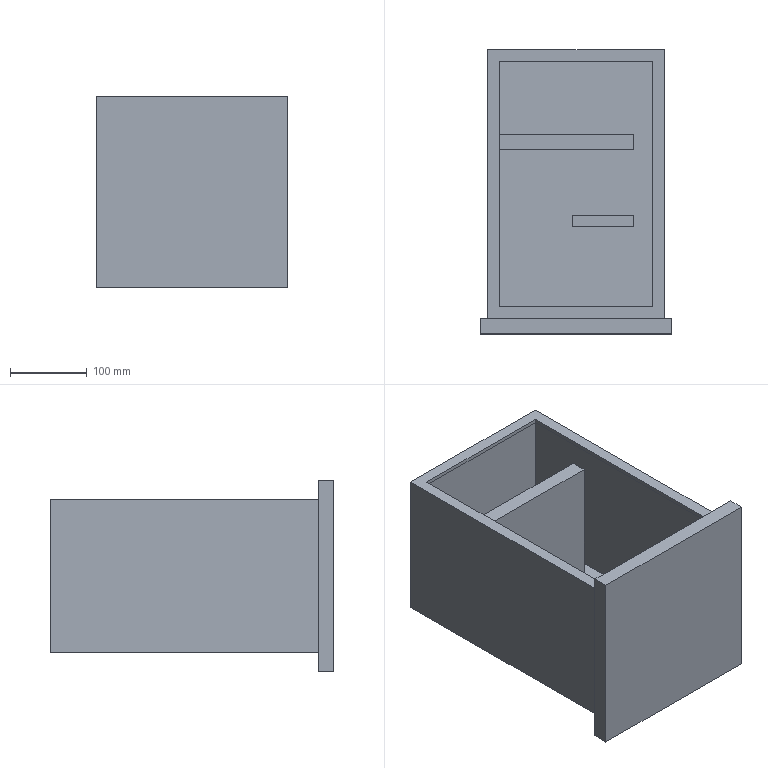Component | SolidWorks | ElectricalCabinet-2 | 1 solid | 30 faces | box 250 x 370 x 250 mm | volume 4917500 mm3 | plane 30
build123d program:
from build123d import *

# Parameters (mm, degrees)
SKETCH1_W           = 350
SKETCH1_H           = 200
BOSS_EXTRUDE1_DEPTH = 230
SHELL1_T            = -10
SKETCH2_W           = 350
SKETCH2_H           = 230
SKETCH2_W_2         = 320
SKETCH2_H_2         = 200
BOSS_EXTRUDE2_DEPTH = 5
SKETCH3_W           = 250
SKETCH3_H           = 250
BOSS_EXTRUDE3_DEPTH = 20
SKETCH4_W           = 20
SKETCH4_H           = 180
BOSS_EXTRUDE4_DEPTH = 180
SKETCH5_W           = 15
SKETCH5_H           = 80
BOSS_EXTRUDE5_DEPTH = 50


with BuildPart() as part:
    # Sketch1 → Boss-Extrude1 (new body)
    with BuildSketch(Plane.XY):
        with Locations((175, 0)):
            Rectangle(SKETCH1_W, SKETCH1_H)
    extrude(amount=BOSS_EXTRUDE1_DEPTH)

    # Shell1
    shell1_openings = [part.faces().sort_by_distance(p)[0] for p in [
        (175, -100, 115),
    ]]
    offset(amount=SHELL1_T, openings=shell1_openings, kind=Kind.INTERSECTION)

    # Sketch2 → Boss-Extrude2 (add)
    with BuildSketch(Plane.XZ.offset(100)):
        with Locations((175, 115)):
            Rectangle(SKETCH2_W, SKETCH2_H)
        with Locations((175, 115)):
            Rectangle(SKETCH2_W_2, SKETCH2_H_2, mode=Mode.SUBTRACT)
    extrude(amount=-BOSS_EXTRUDE2_DEPTH)

    # Sketch3 → Boss-Extrude3 (add)
    with BuildSketch(Plane.ZY):
        with Locations((115, 0)):
            Rectangle(SKETCH3_W, SKETCH3_H)
    extrude(amount=BOSS_EXTRUDE3_DEPTH)

    # Sketch4 → Boss-Extrude4 (add)
    with BuildSketch(Plane.XZ.offset(-90)):
        with Locations((230, 130)):
            Rectangle(SKETCH4_W, SKETCH4_H)
    extrude(amount=BOSS_EXTRUDE4_DEPTH)

    # Sketch5 → Boss-Extrude5 (add)
    with BuildSketch(Plane.XZ.offset(-90)):
        with Locations((127.5, 80)):
            Rectangle(SKETCH5_W, SKETCH5_H)
    extrude(amount=BOSS_EXTRUDE5_DEPTH)


solid = part.part

# Placed as in the assembly
solid = solid.moved(Location((-690, 20, -10), (-90, -90, 0)))
STEP:
#1=COLOUR_RGB('',0.7922,0.8196,0.9333);
#2=FILL_AREA_STYLE_COLOUR('',#1);
#3=FILL_AREA_STYLE('',(#2));
#4=SURFACE_STYLE_FILL_AREA(#3);
#5=SURFACE_SIDE_STYLE('',(#4));
#6=SURFACE_STYLE_USAGE(.BOTH.,#5);
#7=PRESENTATION_STYLE_ASSIGNMENT((#6));
#8=CARTESIAN_POINT('',(-35.827,14.173,-3.937));
#9=VERTEX_POINT('',#8);
#10=CARTESIAN_POINT('',(-35.827,10.236,-3.937));
#11=VERTEX_POINT('',#10);
#12=CARTESIAN_POINT('',(-35.827,0.7874,-3.937));
#13=DIRECTION('',(0.,-1.,0.));
#14=VECTOR('',#13,39.37);
#15=LINE('',#12,#14);
#16=EDGE_CURVE('',#9,#11,#15,.T.);
#17=ORIENTED_EDGE('',*,*,#16,.T.);
#18=CARTESIAN_POINT('',(-28.74,10.236,-3.937));
#19=VERTEX_POINT('',#18);
#20=CARTESIAN_POINT('',(-35.827,10.236,-3.937));
#21=DIRECTION('',(-1.,-0.,0.));
#22=VECTOR('',#21,39.37);
#23=LINE('',#20,#22);
#24=EDGE_CURVE('',#19,#11,#23,.T.);
#25=ORIENTED_EDGE('',*,*,#24,.F.);
#26=CARTESIAN_POINT('',(-28.74,9.449,-3.937));
#27=VERTEX_POINT('',#26);
#28=CARTESIAN_POINT('',(-28.74,10.236,-3.937));
#29=DIRECTION('',(0.,1.,0.));
#30=VECTOR('',#29,39.37);
#31=LINE('',#28,#30);
#32=EDGE_CURVE('',#27,#19,#31,.T.);
#33=ORIENTED_EDGE('',*,*,#32,.F.);
#34=CARTESIAN_POINT('',(-35.827,9.449,-3.937));
#35=VERTEX_POINT('',#34);
#36=CARTESIAN_POINT('',(-35.827,9.449,-3.937));
#37=DIRECTION('',(1.,0.,0.));
#38=VECTOR('',#37,39.37);
#39=LINE('',#36,#38);
#40=EDGE_CURVE('',#35,#27,#39,.T.);
#41=ORIENTED_EDGE('',*,*,#40,.F.);
#42=CARTESIAN_POINT('',(-35.827,1.181,-3.937));
#43=VERTEX_POINT('',#42);
#44=CARTESIAN_POINT('',(-35.827,0.7874,-3.937));
#45=DIRECTION('',(0.,-1.,0.));
#46=VECTOR('',#45,39.37);
#47=LINE('',#44,#46);
#48=EDGE_CURVE('',#35,#43,#47,.T.);
#49=ORIENTED_EDGE('',*,*,#48,.T.);
#50=CARTESIAN_POINT('',(-27.559,1.181,-3.937));
#51=VERTEX_POINT('',#50);
#52=CARTESIAN_POINT('',(-36.22,1.181,-3.937));
#53=DIRECTION('',(1.,0.,0.));
#54=VECTOR('',#53,39.37);
#55=LINE('',#52,#54);
#56=EDGE_CURVE('',#43,#51,#55,.T.);
#57=ORIENTED_EDGE('',*,*,#56,.T.);
#58=CARTESIAN_POINT('',(-27.559,14.173,-3.937));
#59=VERTEX_POINT('',#58);
#60=CARTESIAN_POINT('',(-27.559,0.7874,-3.937));
#61=DIRECTION('',(0.,-1.,0.));
#62=VECTOR('',#61,39.37);
#63=LINE('',#60,#62);
#64=EDGE_CURVE('',#59,#51,#63,.T.);
#65=ORIENTED_EDGE('',*,*,#64,.F.);
#66=CARTESIAN_POINT('',(-36.22,14.173,-3.937));
#67=DIRECTION('',(1.,0.,0.));
#68=VECTOR('',#67,39.37);
#69=LINE('',#66,#68);
#70=EDGE_CURVE('',#9,#59,#69,.T.);
#71=ORIENTED_EDGE('',*,*,#70,.F.);
#72=EDGE_LOOP('',(#17,#25,#33,#41,#49,#57,#65,#71));
#73=FACE_OUTER_BOUND('',#72,.T.);
#74=CARTESIAN_POINT('',(-31.89,6.102,-3.937));
#75=VERTEX_POINT('',#74);
#76=CARTESIAN_POINT('',(-31.89,5.512,-3.937));
#77=VERTEX_POINT('',#76);
#78=CARTESIAN_POINT('',(-31.89,6.102,-3.937));
#79=DIRECTION('',(-0.,-1.,0.));
#80=VECTOR('',#79,39.37);
#81=LINE('',#78,#80);
#82=EDGE_CURVE('',#75,#77,#81,.T.);
#83=ORIENTED_EDGE('',*,*,#82,.F.);
#84=CARTESIAN_POINT('',(-28.74,6.102,-3.937));
#85=VERTEX_POINT('',#84);
#86=CARTESIAN_POINT('',(-28.74,6.102,-3.937));
#87=DIRECTION('',(-1.,0.,0.));
#88=VECTOR('',#87,39.37);
#89=LINE('',#86,#88);
#90=EDGE_CURVE('',#85,#75,#89,.T.);
#91=ORIENTED_EDGE('',*,*,#90,.F.);
#92=CARTESIAN_POINT('',(-28.74,5.512,-3.937));
#93=VERTEX_POINT('',#92);
#94=CARTESIAN_POINT('',(-28.74,6.102,-3.937));
#95=DIRECTION('',(0.,1.,0.));
#96=VECTOR('',#95,39.37);
#97=LINE('',#94,#96);
#98=EDGE_CURVE('',#93,#85,#97,.T.);
#99=ORIENTED_EDGE('',*,*,#98,.F.);
#100=CARTESIAN_POINT('',(-28.74,5.512,-3.937));
#101=DIRECTION('',(1.,0.,0.));
#102=VECTOR('',#101,39.37);
#103=LINE('',#100,#102);
#104=EDGE_CURVE('',#77,#93,#103,.T.);
#105=ORIENTED_EDGE('',*,*,#104,.F.);
#106=EDGE_LOOP('',(#83,#91,#99,#105));
#107=FACE_BOUND('',#106,.T.);
#108=CARTESIAN_POINT('',(-36.22,0.7874,-3.937));
#109=DIRECTION('',(0.,0.,1.));
#110=DIRECTION('',(1.,0.,0.));
#111=AXIS2_PLACEMENT_3D('',#108,#109,#110);
#112=PLANE('',#111);
#113=ADVANCED_FACE('',(#73,#107),#112,.T.);
#114=CARTESIAN_POINT('',(-35.827,10.236,3.15));
#115=VERTEX_POINT('',#114);
#116=CARTESIAN_POINT('',(-35.827,10.236,3.15));
#117=DIRECTION('',(0.,0.,-1.));
#118=VECTOR('',#117,39.37);
#119=LINE('',#116,#118);
#120=EDGE_CURVE('',#115,#11,#119,.T.);
#121=ORIENTED_EDGE('',*,*,#120,.T.);
#122=ORIENTED_EDGE('',*,*,#16,.F.);
#123=CARTESIAN_POINT('',(-35.827,14.173,3.346));
#124=VERTEX_POINT('',#123);
#125=CARTESIAN_POINT('',(-35.827,14.173,-4.331));
#126=DIRECTION('',(0.,0.,-1.));
#127=VECTOR('',#126,39.37);
#128=LINE('',#125,#127);
#129=EDGE_CURVE('',#124,#9,#128,.T.);
#130=ORIENTED_EDGE('',*,*,#129,.F.);
#131=CARTESIAN_POINT('',(-35.827,1.181,3.346));
#132=VERTEX_POINT('',#131);
#133=CARTESIAN_POINT('',(-35.827,0.7874,3.346));
#134=DIRECTION('',(0.,-1.,0.));
#135=VECTOR('',#134,39.37);
#136=LINE('',#133,#135);
#137=EDGE_CURVE('',#124,#132,#136,.T.);
#138=ORIENTED_EDGE('',*,*,#137,.T.);
#139=CARTESIAN_POINT('',(-35.827,1.181,-4.331));
#140=DIRECTION('',(0.,0.,1.));
#141=VECTOR('',#140,39.37);
#142=LINE('',#139,#141);
#143=EDGE_CURVE('',#43,#132,#142,.T.);
#144=ORIENTED_EDGE('',*,*,#143,.F.);
#145=ORIENTED_EDGE('',*,*,#48,.F.);
#146=CARTESIAN_POINT('',(-35.827,9.449,3.15));
#147=VERTEX_POINT('',#146);
#148=CARTESIAN_POINT('',(-35.827,9.449,3.15));
#149=DIRECTION('',(0.,0.,-1.));
#150=VECTOR('',#149,39.37);
#151=LINE('',#148,#150);
#152=EDGE_CURVE('',#147,#35,#151,.T.);
#153=ORIENTED_EDGE('',*,*,#152,.F.);
#154=CARTESIAN_POINT('',(-35.827,10.236,3.15));
#155=DIRECTION('',(0.,-1.,0.));
#156=VECTOR('',#155,39.37);
#157=LINE('',#154,#156);
#158=EDGE_CURVE('',#115,#147,#157,.T.);
#159=ORIENTED_EDGE('',*,*,#158,.F.);
#160=EDGE_LOOP('',(#121,#122,#130,#138,#144,#145,#153,#159));
#161=FACE_OUTER_BOUND('',#160,.T.);
#162=CARTESIAN_POINT('',(-35.827,0.7874,-0.3937));
#163=DIRECTION('',(-1.,0.,0.));
#164=DIRECTION('',(0.,1.,0.));
#165=AXIS2_PLACEMENT_3D('',#162,#163,#164);
#166=PLANE('',#165);
#167=ADVANCED_FACE('',(#161),#166,.F.);
#168=CARTESIAN_POINT('',(-27.165,0.7874,3.543));
#169=VERTEX_POINT('',#168);
#170=CARTESIAN_POINT('',(-27.165,14.567,3.543));
#171=VERTEX_POINT('',#170);
#172=CARTESIAN_POINT('',(-27.165,0.7874,3.543));
#173=DIRECTION('',(0.,1.,0.));
#174=VECTOR('',#173,39.37);
#175=LINE('',#172,#174);
#176=EDGE_CURVE('',#169,#171,#175,.T.);
#177=ORIENTED_EDGE('',*,*,#176,.T.);
#178=CARTESIAN_POINT('',(-36.22,14.567,3.543));
#179=VERTEX_POINT('',#178);
#180=CARTESIAN_POINT('',(-36.22,14.567,3.543));
#181=DIRECTION('',(1.,0.,0.));
#182=VECTOR('',#181,39.37);
#183=LINE('',#180,#182);
#184=EDGE_CURVE('',#179,#171,#183,.T.);
#185=ORIENTED_EDGE('',*,*,#184,.F.);
#186=CARTESIAN_POINT('',(-36.22,0.7874,3.543));
#187=VERTEX_POINT('',#186);
#188=CARTESIAN_POINT('',(-36.22,0.7874,3.543));
#189=DIRECTION('',(0.,1.,0.));
#190=VECTOR('',#189,39.37);
#191=LINE('',#188,#190);
#192=EDGE_CURVE('',#187,#179,#191,.T.);
#193=ORIENTED_EDGE('',*,*,#192,.F.);
#194=CARTESIAN_POINT('',(-36.22,0.7874,3.543));
#195=DIRECTION('',(1.,0.,0.));
#196=VECTOR('',#195,39.37);
#197=LINE('',#194,#196);
#198=EDGE_CURVE('',#187,#169,#197,.T.);
#199=ORIENTED_EDGE('',*,*,#198,.T.);
#200=EDGE_LOOP('',(#177,#185,#193,#199));
#201=FACE_OUTER_BOUND('',#200,.T.);
#202=CARTESIAN_POINT('',(-35.63,1.378,3.543));
#203=VERTEX_POINT('',#202);
#204=CARTESIAN_POINT('',(-27.756,1.378,3.543));
#205=VERTEX_POINT('',#204);
#206=CARTESIAN_POINT('',(-35.63,1.378,3.543));
#207=DIRECTION('',(1.,-0.,0.));
#208=VECTOR('',#207,39.37);
#209=LINE('',#206,#208);
#210=EDGE_CURVE('',#203,#205,#209,.T.);
#211=ORIENTED_EDGE('',*,*,#210,.F.);
#212=CARTESIAN_POINT('',(-35.63,13.976,3.543));
#213=VERTEX_POINT('',#212);
#214=CARTESIAN_POINT('',(-35.63,13.976,3.543));
#215=DIRECTION('',(0.,-1.,0.));
#216=VECTOR('',#215,39.37);
#217=LINE('',#214,#216);
#218=EDGE_CURVE('',#213,#203,#217,.T.);
#219=ORIENTED_EDGE('',*,*,#218,.F.);
#220=CARTESIAN_POINT('',(-27.756,13.976,3.543));
#221=VERTEX_POINT('',#220);
#222=CARTESIAN_POINT('',(-35.63,13.976,3.543));
#223=DIRECTION('',(-1.,0.,0.));
#224=VECTOR('',#223,39.37);
#225=LINE('',#222,#224);
#226=EDGE_CURVE('',#221,#213,#225,.T.);
#227=ORIENTED_EDGE('',*,*,#226,.F.);
#228=CARTESIAN_POINT('',(-27.756,13.976,3.543));
#229=DIRECTION('',(-0.,1.,0.));
#230=VECTOR('',#229,39.37);
#231=LINE('',#228,#230);
#232=EDGE_CURVE('',#205,#221,#231,.T.);
#233=ORIENTED_EDGE('',*,*,#232,.F.);
#234=EDGE_LOOP('',(#211,#219,#227,#233));
#235=FACE_BOUND('',#234,.T.);
#236=CARTESIAN_POINT('',(-36.22,0.7874,3.543));
#237=DIRECTION('',(0.,0.,-1.));
#238=DIRECTION('',(-1.,0.,0.));
#239=AXIS2_PLACEMENT_3D('',#236,#237,#238);
#240=PLANE('',#239);
#241=ADVANCED_FACE('',(#201,#235),#240,.F.);
#242=CARTESIAN_POINT('',(-36.22,14.567,-4.331));
#243=VERTEX_POINT('',#242);
#244=CARTESIAN_POINT('',(-27.165,14.567,-4.331));
#245=VERTEX_POINT('',#244);
#246=CARTESIAN_POINT('',(-36.22,14.567,-4.331));
#247=DIRECTION('',(1.,0.,0.));
#248=VECTOR('',#247,39.37);
#249=LINE('',#246,#248);
#250=EDGE_CURVE('',#243,#245,#249,.T.);
#251=ORIENTED_EDGE('',*,*,#250,.F.);
#252=CARTESIAN_POINT('',(-36.22,14.567,-4.331));
#253=DIRECTION('',(0.,0.,-1.));
#254=VECTOR('',#253,39.37);
#255=LINE('',#252,#254);
#256=EDGE_CURVE('',#179,#243,#255,.T.);
#257=ORIENTED_EDGE('',*,*,#256,.F.);
#258=ORIENTED_EDGE('',*,*,#184,.T.);
#259=CARTESIAN_POINT('',(-27.165,14.567,-4.331));
#260=DIRECTION('',(0.,0.,-1.));
#261=VECTOR('',#260,39.37);
#262=LINE('',#259,#261);
#263=EDGE_CURVE('',#171,#245,#262,.T.);
#264=ORIENTED_EDGE('',*,*,#263,.T.);
#265=EDGE_LOOP('',(#251,#257,#258,#264));
#266=FACE_OUTER_BOUND('',#265,.T.);
#267=CARTESIAN_POINT('',(-36.22,14.567,-4.331));
#268=DIRECTION('',(0.,-1.,0.));
#269=DIRECTION('',(-1.,0.,0.));
#270=AXIS2_PLACEMENT_3D('',#267,#268,#269);
#271=PLANE('',#270);
#272=ADVANCED_FACE('',(#266),#271,.F.);
#273=CARTESIAN_POINT('',(-27.165,0.7874,-4.331));
#274=VERTEX_POINT('',#273);
#275=CARTESIAN_POINT('',(-27.165,0.7874,-4.331));
#276=DIRECTION('',(0.,-1.,0.));
#277=VECTOR('',#276,39.37);
#278=LINE('',#275,#277);
#279=EDGE_CURVE('',#245,#274,#278,.T.);
#280=ORIENTED_EDGE('',*,*,#279,.T.);
#281=CARTESIAN_POINT('',(-36.22,0.7874,-4.331));
#282=VERTEX_POINT('',#281);
#283=CARTESIAN_POINT('',(-36.22,0.7874,-4.331));
#284=DIRECTION('',(1.,0.,0.));
#285=VECTOR('',#284,39.37);
#286=LINE('',#283,#285);
#287=EDGE_CURVE('',#282,#274,#286,.T.);
#288=ORIENTED_EDGE('',*,*,#287,.F.);
#289=CARTESIAN_POINT('',(-36.22,0.7874,-4.331));
#290=DIRECTION('',(0.,-1.,0.));
#291=VECTOR('',#290,39.37);
#292=LINE('',#289,#291);
#293=EDGE_CURVE('',#243,#282,#292,.T.);
#294=ORIENTED_EDGE('',*,*,#293,.F.);
#295=ORIENTED_EDGE('',*,*,#250,.T.);
#296=EDGE_LOOP('',(#280,#288,#294,#295));
#297=FACE_OUTER_BOUND('',#296,.T.);
#298=CARTESIAN_POINT('',(-36.22,0.7874,-4.331));
#299=DIRECTION('',(0.,0.,1.));
#300=DIRECTION('',(1.,0.,0.));
#301=AXIS2_PLACEMENT_3D('',#298,#299,#300);
#302=PLANE('',#301);
#303=ADVANCED_FACE('',(#297),#302,.F.);
#304=CARTESIAN_POINT('',(-36.22,0.7874,-4.331));
#305=DIRECTION('',(0.,0.,1.));
#306=VECTOR('',#305,39.37);
#307=LINE('',#304,#306);
#308=EDGE_CURVE('',#282,#187,#307,.T.);
#309=ORIENTED_EDGE('',*,*,#308,.T.);
#310=ORIENTED_EDGE('',*,*,#192,.T.);
#311=ORIENTED_EDGE('',*,*,#256,.T.);
#312=ORIENTED_EDGE('',*,*,#293,.T.);
#313=EDGE_LOOP('',(#309,#310,#311,#312));
#314=FACE_OUTER_BOUND('',#313,.T.);
#315=CARTESIAN_POINT('',(-36.22,0.7874,-0.3937));
#316=DIRECTION('',(-1.,0.,0.));
#317=DIRECTION('',(0.,1.,0.));
#318=AXIS2_PLACEMENT_3D('',#315,#316,#317);
#319=PLANE('',#318);
#320=ADVANCED_FACE('',(#314),#319,.T.);
#321=ORIENTED_EDGE('',*,*,#279,.F.);
#322=ORIENTED_EDGE('',*,*,#263,.F.);
#323=ORIENTED_EDGE('',*,*,#176,.F.);
#324=CARTESIAN_POINT('',(-27.165,0.7874,-4.331));
#325=DIRECTION('',(0.,0.,1.));
#326=VECTOR('',#325,39.37);
#327=LINE('',#324,#326);
#328=EDGE_CURVE('',#274,#169,#327,.T.);
#329=ORIENTED_EDGE('',*,*,#328,.F.);
#330=EDGE_LOOP('',(#321,#322,#323,#329));
#331=FACE_OUTER_BOUND('',#330,.T.);
#332=CARTESIAN_POINT('',(-27.165,0.7874,-0.3937));
#333=DIRECTION('',(-1.,0.,0.));
#334=DIRECTION('',(0.,1.,0.));
#335=AXIS2_PLACEMENT_3D('',#332,#333,#334);
#336=PLANE('',#335);
#337=ADVANCED_FACE('',(#331),#336,.F.);
#338=CARTESIAN_POINT('',(-35.63,13.976,3.346));
#339=VERTEX_POINT('',#338);
#340=CARTESIAN_POINT('',(-35.63,1.378,3.346));
#341=VERTEX_POINT('',#340);
#342=CARTESIAN_POINT('',(-35.63,13.976,3.346));
#343=DIRECTION('',(0.,-1.,0.));
#344=VECTOR('',#343,39.37);
#345=LINE('',#342,#344);
#346=EDGE_CURVE('',#339,#341,#345,.T.);
#347=ORIENTED_EDGE('',*,*,#346,.T.);
#348=CARTESIAN_POINT('',(-27.756,1.378,3.346));
#349=VERTEX_POINT('',#348);
#350=CARTESIAN_POINT('',(-35.63,1.378,3.346));
#351=DIRECTION('',(1.,-0.,0.));
#352=VECTOR('',#351,39.37);
#353=LINE('',#350,#352);
#354=EDGE_CURVE('',#341,#349,#353,.T.);
#355=ORIENTED_EDGE('',*,*,#354,.T.);
#356=CARTESIAN_POINT('',(-27.756,13.976,3.346));
#357=VERTEX_POINT('',#356);
#358=CARTESIAN_POINT('',(-27.756,13.976,3.346));
#359=DIRECTION('',(-0.,1.,0.));
#360=VECTOR('',#359,39.37);
#361=LINE('',#358,#360);
#362=EDGE_CURVE('',#349,#357,#361,.T.);
#363=ORIENTED_EDGE('',*,*,#362,.T.);
#364=CARTESIAN_POINT('',(-35.63,13.976,3.346));
#365=DIRECTION('',(-1.,0.,0.));
#366=VECTOR('',#365,39.37);
#367=LINE('',#364,#366);
#368=EDGE_CURVE('',#357,#339,#367,.T.);
#369=ORIENTED_EDGE('',*,*,#368,.T.);
#370=EDGE_LOOP('',(#347,#355,#363,#369));
#371=FACE_BOUND('',#370,.T.);
#372=ORIENTED_EDGE('',*,*,#137,.F.);
#373=CARTESIAN_POINT('',(-27.559,14.173,3.346));
#374=VERTEX_POINT('',#373);
#375=CARTESIAN_POINT('',(-36.22,14.173,3.346));
#376=DIRECTION('',(1.,0.,0.));
#377=VECTOR('',#376,39.37);
#378=LINE('',#375,#377);
#379=EDGE_CURVE('',#124,#374,#378,.T.);
#380=ORIENTED_EDGE('',*,*,#379,.T.);
#381=CARTESIAN_POINT('',(-27.559,1.181,3.346));
#382=VERTEX_POINT('',#381);
#383=CARTESIAN_POINT('',(-27.559,0.7874,3.346));
#384=DIRECTION('',(0.,-1.,0.));
#385=VECTOR('',#384,39.37);
#386=LINE('',#383,#385);
#387=EDGE_CURVE('',#374,#382,#386,.T.);
#388=ORIENTED_EDGE('',*,*,#387,.T.);
#389=CARTESIAN_POINT('',(-36.22,1.181,3.346));
#390=DIRECTION('',(-1.,0.,0.));
#391=VECTOR('',#390,39.37);
#392=LINE('',#389,#391);
#393=EDGE_CURVE('',#382,#132,#392,.T.);
#394=ORIENTED_EDGE('',*,*,#393,.T.);
#395=EDGE_LOOP('',(#372,#380,#388,#394));
#396=FACE_OUTER_BOUND('',#395,.T.);
#397=CARTESIAN_POINT('',(-27.165,0.7874,3.346));
#398=DIRECTION('',(0.,0.,-1.));
#399=DIRECTION('',(-1.,0.,0.));
#400=AXIS2_PLACEMENT_3D('',#397,#398,#399);
#401=PLANE('',#400);
#402=ADVANCED_FACE('',(#371,#396),#401,.T.);
#403=ORIENTED_EDGE('',*,*,#218,.T.);
#404=CARTESIAN_POINT('',(-35.63,1.378,3.346));
#405=DIRECTION('',(0.,0.,1.));
#406=VECTOR('',#405,39.37);
#407=LINE('',#404,#406);
#408=EDGE_CURVE('',#341,#203,#407,.T.);
#409=ORIENTED_EDGE('',*,*,#408,.F.);
#410=ORIENTED_EDGE('',*,*,#346,.F.);
#411=CARTESIAN_POINT('',(-35.63,13.976,3.346));
#412=DIRECTION('',(0.,0.,1.));
#413=VECTOR('',#412,39.37);
#414=LINE('',#411,#413);
#415=EDGE_CURVE('',#339,#213,#414,.T.);
#416=ORIENTED_EDGE('',*,*,#415,.T.);
#417=EDGE_LOOP('',(#403,#409,#410,#416));
#418=FACE_OUTER_BOUND('',#417,.T.);
#419=CARTESIAN_POINT('',(-35.63,13.976,3.346));
#420=DIRECTION('',(-1.,0.,0.));
#421=DIRECTION('',(0.,1.,0.));
#422=AXIS2_PLACEMENT_3D('',#419,#420,#421);
#423=PLANE('',#422);
#424=ADVANCED_FACE('',(#418),#423,.F.);
#425=ORIENTED_EDGE('',*,*,#226,.T.);
#426=ORIENTED_EDGE('',*,*,#415,.F.);
#427=ORIENTED_EDGE('',*,*,#368,.F.);
#428=CARTESIAN_POINT('',(-27.756,13.976,3.346));
#429=DIRECTION('',(0.,0.,1.));
#430=VECTOR('',#429,39.37);
#431=LINE('',#428,#430);
#432=EDGE_CURVE('',#357,#221,#431,.T.);
#433=ORIENTED_EDGE('',*,*,#432,.T.);
#434=EDGE_LOOP('',(#425,#426,#427,#433));
#435=FACE_OUTER_BOUND('',#434,.T.);
#436=CARTESIAN_POINT('',(-35.63,13.976,3.346));
#437=DIRECTION('',(0.,1.,0.));
#438=DIRECTION('',(1.,0.,0.));
#439=AXIS2_PLACEMENT_3D('',#436,#437,#438);
#440=PLANE('',#439);
#441=ADVANCED_FACE('',(#435),#440,.F.);
#442=ORIENTED_EDGE('',*,*,#232,.T.);
#443=ORIENTED_EDGE('',*,*,#432,.F.);
#444=ORIENTED_EDGE('',*,*,#362,.F.);
#445=CARTESIAN_POINT('',(-27.756,1.378,3.346));
#446=DIRECTION('',(0.,0.,1.));
#447=VECTOR('',#446,39.37);
#448=LINE('',#445,#447);
#449=EDGE_CURVE('',#349,#205,#448,.T.);
#450=ORIENTED_EDGE('',*,*,#449,.T.);
#451=EDGE_LOOP('',(#442,#443,#444,#450));
#452=FACE_OUTER_BOUND('',#451,.T.);
#453=CARTESIAN_POINT('',(-27.756,13.976,3.346));
#454=DIRECTION('',(1.,0.,0.));
#455=DIRECTION('',(0.,-1.,0.));
#456=AXIS2_PLACEMENT_3D('',#453,#454,#455);
#457=PLANE('',#456);
#458=ADVANCED_FACE('',(#452),#457,.F.);
#459=ORIENTED_EDGE('',*,*,#210,.T.);
#460=ORIENTED_EDGE('',*,*,#449,.F.);
#461=ORIENTED_EDGE('',*,*,#354,.F.);
#462=ORIENTED_EDGE('',*,*,#408,.T.);
#463=EDGE_LOOP('',(#459,#460,#461,#462));
#464=FACE_OUTER_BOUND('',#463,.T.);
#465=CARTESIAN_POINT('',(-35.63,1.378,3.346));
#466=DIRECTION('',(-0.,-1.,0.));
#467=DIRECTION('',(-1.,0.,0.));
#468=AXIS2_PLACEMENT_3D('',#465,#466,#467);
#469=PLANE('',#468);
#470=ADVANCED_FACE('',(#464),#469,.F.);
#471=ORIENTED_EDGE('',*,*,#387,.F.);
#472=CARTESIAN_POINT('',(-27.559,14.173,-4.331));
#473=DIRECTION('',(0.,0.,-1.));
#474=VECTOR('',#473,39.37);
#475=LINE('',#472,#474);
#476=EDGE_CURVE('',#374,#59,#475,.T.);
#477=ORIENTED_EDGE('',*,*,#476,.T.);
#478=ORIENTED_EDGE('',*,*,#64,.T.);
#479=CARTESIAN_POINT('',(-27.559,1.181,-4.331));
#480=DIRECTION('',(0.,0.,1.));
#481=VECTOR('',#480,39.37);
#482=LINE('',#479,#481);
#483=EDGE_CURVE('',#51,#382,#482,.T.);
#484=ORIENTED_EDGE('',*,*,#483,.T.);
#485=EDGE_LOOP('',(#471,#477,#478,#484));
#486=FACE_OUTER_BOUND('',#485,.T.);
#487=CARTESIAN_POINT('',(-27.559,0.7874,-0.3937));
#488=DIRECTION('',(-1.,0.,0.));
#489=DIRECTION('',(0.,1.,0.));
#490=AXIS2_PLACEMENT_3D('',#487,#488,#489);
#491=PLANE('',#490);
#492=ADVANCED_FACE('',(#486),#491,.T.);
#493=ORIENTED_EDGE('',*,*,#379,.F.);
#494=ORIENTED_EDGE('',*,*,#129,.T.);
#495=ORIENTED_EDGE('',*,*,#70,.T.);
#496=ORIENTED_EDGE('',*,*,#476,.F.);
#497=EDGE_LOOP('',(#493,#494,#495,#496));
#498=FACE_OUTER_BOUND('',#497,.T.);
#499=CARTESIAN_POINT('',(-36.22,14.173,-4.331));
#500=DIRECTION('',(0.,-1.,0.));
#501=DIRECTION('',(-1.,0.,0.));
#502=AXIS2_PLACEMENT_3D('',#499,#500,#501);
#503=PLANE('',#502);
#504=ADVANCED_FACE('',(#498),#503,.T.);
#505=ORIENTED_EDGE('',*,*,#393,.F.);
#506=ORIENTED_EDGE('',*,*,#483,.F.);
#507=ORIENTED_EDGE('',*,*,#56,.F.);
#508=ORIENTED_EDGE('',*,*,#143,.T.);
#509=EDGE_LOOP('',(#505,#506,#507,#508));
#510=FACE_OUTER_BOUND('',#509,.T.);
#511=CARTESIAN_POINT('',(-36.22,1.181,-4.331));
#512=DIRECTION('',(0.,1.,0.));
#513=DIRECTION('',(1.,0.,0.));
#514=AXIS2_PLACEMENT_3D('',#511,#512,#513);
#515=PLANE('',#514);
#516=ADVANCED_FACE('',(#510),#515,.T.);
#517=CARTESIAN_POINT('',(-36.614,0.7874,4.528));
#518=VERTEX_POINT('',#517);
#519=CARTESIAN_POINT('',(-36.614,0.7874,-5.315));
#520=VERTEX_POINT('',#519);
#521=CARTESIAN_POINT('',(-36.614,0.7874,4.528));
#522=DIRECTION('',(0.,0.,-1.));
#523=VECTOR('',#522,39.37);
#524=LINE('',#521,#523);
#525=EDGE_CURVE('',#518,#520,#524,.T.);
#526=ORIENTED_EDGE('',*,*,#525,.F.);
#527=CARTESIAN_POINT('',(-26.772,0.7874,4.528));
#528=VERTEX_POINT('',#527);
#529=CARTESIAN_POINT('',(-36.614,0.7874,4.528));
#530=DIRECTION('',(-1.,0.,0.));
#531=VECTOR('',#530,39.37);
#532=LINE('',#529,#531);
#533=EDGE_CURVE('',#528,#518,#532,.T.);
#534=ORIENTED_EDGE('',*,*,#533,.F.);
#535=CARTESIAN_POINT('',(-26.772,0.7874,-5.315));
#536=VERTEX_POINT('',#535);
#537=CARTESIAN_POINT('',(-26.772,0.7874,4.528));
#538=DIRECTION('',(-0.,0.,1.));
#539=VECTOR('',#538,39.37);
#540=LINE('',#537,#539);
#541=EDGE_CURVE('',#536,#528,#540,.T.);
#542=ORIENTED_EDGE('',*,*,#541,.F.);
#543=CARTESIAN_POINT('',(-36.614,0.7874,-5.315));
#544=DIRECTION('',(1.,0.,-0.));
#545=VECTOR('',#544,39.37);
#546=LINE('',#543,#545);
#547=EDGE_CURVE('',#520,#536,#546,.T.);
#548=ORIENTED_EDGE('',*,*,#547,.F.);
#549=EDGE_LOOP('',(#526,#534,#542,#548));
#550=FACE_OUTER_BOUND('',#549,.T.);
#551=ORIENTED_EDGE('',*,*,#287,.T.);
#552=ORIENTED_EDGE('',*,*,#328,.T.);
#553=ORIENTED_EDGE('',*,*,#198,.F.);
#554=ORIENTED_EDGE('',*,*,#308,.F.);
#555=EDGE_LOOP('',(#551,#552,#553,#554));
#556=FACE_BOUND('',#555,.T.);
#557=CARTESIAN_POINT('',(-27.165,0.7874,-0.3937));
#558=DIRECTION('',(0.,-1.,0.));
#559=DIRECTION('',(-1.,0.,0.));
#560=AXIS2_PLACEMENT_3D('',#557,#558,#559);
#561=PLANE('',#560);
#562=ADVANCED_FACE('',(#550,#556),#561,.F.);
#563=ORIENTED_EDGE('',*,*,#525,.T.);
#564=CARTESIAN_POINT('',(-36.614,0.,-5.315));
#565=VERTEX_POINT('',#564);
#566=CARTESIAN_POINT('',(-36.614,0.,-5.315));
#567=DIRECTION('',(0.,1.,0.));
#568=VECTOR('',#567,39.37);
#569=LINE('',#566,#568);
#570=EDGE_CURVE('',#565,#520,#569,.T.);
#571=ORIENTED_EDGE('',*,*,#570,.F.);
#572=CARTESIAN_POINT('',(-36.614,0.,4.528));
#573=VERTEX_POINT('',#572);
#574=CARTESIAN_POINT('',(-36.614,0.,4.528));
#575=DIRECTION('',(0.,0.,-1.));
#576=VECTOR('',#575,39.37);
#577=LINE('',#574,#576);
#578=EDGE_CURVE('',#573,#565,#577,.T.);
#579=ORIENTED_EDGE('',*,*,#578,.F.);
#580=CARTESIAN_POINT('',(-36.614,0.,4.528));
#581=DIRECTION('',(0.,1.,0.));
#582=VECTOR('',#581,39.37);
#583=LINE('',#580,#582);
#584=EDGE_CURVE('',#573,#518,#583,.T.);
#585=ORIENTED_EDGE('',*,*,#584,.T.);
#586=EDGE_LOOP('',(#563,#571,#579,#585));
#587=FACE_OUTER_BOUND('',#586,.T.);
#588=CARTESIAN_POINT('',(-36.614,0.,4.528));
#589=DIRECTION('',(1.,0.,0.));
#590=DIRECTION('',(0.,-1.,0.));
#591=AXIS2_PLACEMENT_3D('',#588,#589,#590);
#592=PLANE('',#591);
#593=ADVANCED_FACE('',(#587),#592,.F.);
#594=ORIENTED_EDGE('',*,*,#547,.T.);
#595=CARTESIAN_POINT('',(-26.772,0.,-5.315));
#596=VERTEX_POINT('',#595);
#597=CARTESIAN_POINT('',(-26.772,0.,-5.315));
#598=DIRECTION('',(0.,1.,0.));
#599=VECTOR('',#598,39.37);
#600=LINE('',#597,#599);
#601=EDGE_CURVE('',#596,#536,#600,.T.);
#602=ORIENTED_EDGE('',*,*,#601,.F.);
#603=CARTESIAN_POINT('',(-36.614,0.,-5.315));
#604=DIRECTION('',(1.,0.,-0.));
#605=VECTOR('',#604,39.37);
#606=LINE('',#603,#605);
#607=EDGE_CURVE('',#565,#596,#606,.T.);
#608=ORIENTED_EDGE('',*,*,#607,.F.);
#609=ORIENTED_EDGE('',*,*,#570,.T.);
#610=EDGE_LOOP('',(#594,#602,#608,#609));
#611=FACE_OUTER_BOUND('',#610,.T.);
#612=CARTESIAN_POINT('',(-36.614,0.,-5.315));
#613=DIRECTION('',(0.,0.,1.));
#614=DIRECTION('',(1.,0.,-0.));
#615=AXIS2_PLACEMENT_3D('',#612,#613,#614);
#616=PLANE('',#615);
#617=ADVANCED_FACE('',(#611),#616,.F.);
#618=ORIENTED_EDGE('',*,*,#541,.T.);
#619=CARTESIAN_POINT('',(-26.772,0.,4.528));
#620=VERTEX_POINT('',#619);
#621=CARTESIAN_POINT('',(-26.772,0.,4.528));
#622=DIRECTION('',(0.,1.,0.));
#623=VECTOR('',#622,39.37);
#624=LINE('',#621,#623);
#625=EDGE_CURVE('',#620,#528,#624,.T.);
#626=ORIENTED_EDGE('',*,*,#625,.F.);
#627=CARTESIAN_POINT('',(-26.772,0.,4.528));
#628=DIRECTION('',(-0.,0.,1.));
#629=VECTOR('',#628,39.37);
#630=LINE('',#627,#629);
#631=EDGE_CURVE('',#596,#620,#630,.T.);
#632=ORIENTED_EDGE('',*,*,#631,.F.);
#633=ORIENTED_EDGE('',*,*,#601,.T.);
#634=EDGE_LOOP('',(#618,#626,#632,#633));
#635=FACE_OUTER_BOUND('',#634,.T.);
#636=CARTESIAN_POINT('',(-26.772,0.,4.528));
#637=DIRECTION('',(-1.,0.,-0.));
#638=DIRECTION('',(-0.,0.,1.));
#639=AXIS2_PLACEMENT_3D('',#636,#637,#638);
#640=PLANE('',#639);
#641=ADVANCED_FACE('',(#635),#640,.F.);
#642=ORIENTED_EDGE('',*,*,#533,.T.);
#643=ORIENTED_EDGE('',*,*,#584,.F.);
#644=CARTESIAN_POINT('',(-36.614,0.,4.528));
#645=DIRECTION('',(-1.,0.,0.));
#646=VECTOR('',#645,39.37);
#647=LINE('',#644,#646);
#648=EDGE_CURVE('',#620,#573,#647,.T.);
#649=ORIENTED_EDGE('',*,*,#648,.F.);
#650=ORIENTED_EDGE('',*,*,#625,.T.);
#651=EDGE_LOOP('',(#642,#643,#649,#650));
#652=FACE_OUTER_BOUND('',#651,.T.);
#653=CARTESIAN_POINT('',(-36.614,0.,4.528));
#654=DIRECTION('',(-0.,0.,-1.));
#655=DIRECTION('',(-1.,0.,0.));
#656=AXIS2_PLACEMENT_3D('',#653,#654,#655);
#657=PLANE('',#656);
#658=ADVANCED_FACE('',(#652),#657,.F.);
#659=ORIENTED_EDGE('',*,*,#578,.T.);
#660=ORIENTED_EDGE('',*,*,#607,.T.);
#661=ORIENTED_EDGE('',*,*,#631,.T.);
#662=ORIENTED_EDGE('',*,*,#648,.T.);
#663=EDGE_LOOP('',(#659,#660,#661,#662));
#664=FACE_OUTER_BOUND('',#663,.T.);
#665=CARTESIAN_POINT('',(-27.165,0.,-0.3937));
#666=DIRECTION('',(0.,-1.,0.));
#667=DIRECTION('',(-1.,0.,0.));
#668=AXIS2_PLACEMENT_3D('',#665,#666,#667);
#669=PLANE('',#668);
#670=ADVANCED_FACE('',(#664),#669,.T.);
#671=ORIENTED_EDGE('',*,*,#24,.T.);
#672=ORIENTED_EDGE('',*,*,#120,.F.);
#673=CARTESIAN_POINT('',(-28.74,10.236,3.15));
#674=VERTEX_POINT('',#673);
#675=CARTESIAN_POINT('',(-35.827,10.236,3.15));
#676=DIRECTION('',(-1.,-0.,0.));
#677=VECTOR('',#676,39.37);
#678=LINE('',#675,#677);
#679=EDGE_CURVE('',#674,#115,#678,.T.);
#680=ORIENTED_EDGE('',*,*,#679,.F.);
#681=CARTESIAN_POINT('',(-28.74,10.236,3.15));
#682=DIRECTION('',(0.,0.,-1.));
#683=VECTOR('',#682,39.37);
#684=LINE('',#681,#683);
#685=EDGE_CURVE('',#674,#19,#684,.T.);
#686=ORIENTED_EDGE('',*,*,#685,.T.);
#687=EDGE_LOOP('',(#671,#672,#680,#686));
#688=FACE_OUTER_BOUND('',#687,.T.);
#689=CARTESIAN_POINT('',(-35.827,10.236,3.15));
#690=DIRECTION('',(0.,-1.,0.));
#691=DIRECTION('',(-1.,-0.,0.));
#692=AXIS2_PLACEMENT_3D('',#689,#690,#691);
#693=PLANE('',#692);
#694=ADVANCED_FACE('',(#688),#693,.F.);
#695=ORIENTED_EDGE('',*,*,#40,.T.);
#696=CARTESIAN_POINT('',(-28.74,9.449,3.15));
#697=VERTEX_POINT('',#696);
#698=CARTESIAN_POINT('',(-28.74,9.449,3.15));
#699=DIRECTION('',(0.,0.,-1.));
#700=VECTOR('',#699,39.37);
#701=LINE('',#698,#700);
#702=EDGE_CURVE('',#697,#27,#701,.T.);
#703=ORIENTED_EDGE('',*,*,#702,.F.);
#704=CARTESIAN_POINT('',(-35.827,9.449,3.15));
#705=DIRECTION('',(1.,0.,0.));
#706=VECTOR('',#705,39.37);
#707=LINE('',#704,#706);
#708=EDGE_CURVE('',#147,#697,#707,.T.);
#709=ORIENTED_EDGE('',*,*,#708,.F.);
#710=ORIENTED_EDGE('',*,*,#152,.T.);
#711=EDGE_LOOP('',(#695,#703,#709,#710));
#712=FACE_OUTER_BOUND('',#711,.T.);
#713=CARTESIAN_POINT('',(-35.827,9.449,3.15));
#714=DIRECTION('',(-0.,1.,0.));
#715=DIRECTION('',(1.,0.,0.));
#716=AXIS2_PLACEMENT_3D('',#713,#714,#715);
#717=PLANE('',#716);
#718=ADVANCED_FACE('',(#712),#717,.F.);
#719=ORIENTED_EDGE('',*,*,#32,.T.);
#720=ORIENTED_EDGE('',*,*,#685,.F.);
#721=CARTESIAN_POINT('',(-28.74,10.236,3.15));
#722=DIRECTION('',(0.,1.,0.));
#723=VECTOR('',#722,39.37);
#724=LINE('',#721,#723);
#725=EDGE_CURVE('',#697,#674,#724,.T.);
#726=ORIENTED_EDGE('',*,*,#725,.F.);
#727=ORIENTED_EDGE('',*,*,#702,.T.);
#728=EDGE_LOOP('',(#719,#720,#726,#727));
#729=FACE_OUTER_BOUND('',#728,.T.);
#730=CARTESIAN_POINT('',(-28.74,10.236,3.15));
#731=DIRECTION('',(-1.,0.,0.));
#732=DIRECTION('',(0.,1.,0.));
#733=AXIS2_PLACEMENT_3D('',#730,#731,#732);
#734=PLANE('',#733);
#735=ADVANCED_FACE('',(#729),#734,.F.);
#736=ORIENTED_EDGE('',*,*,#679,.T.);
#737=ORIENTED_EDGE('',*,*,#158,.T.);
#738=ORIENTED_EDGE('',*,*,#708,.T.);
#739=ORIENTED_EDGE('',*,*,#725,.T.);
#740=EDGE_LOOP('',(#736,#737,#738,#739));
#741=FACE_OUTER_BOUND('',#740,.T.);
#742=CARTESIAN_POINT('',(-27.165,0.7874,3.15));
#743=DIRECTION('',(0.,0.,-1.));
#744=DIRECTION('',(-1.,0.,0.));
#745=AXIS2_PLACEMENT_3D('',#742,#743,#744);
#746=PLANE('',#745);
#747=ADVANCED_FACE('',(#741),#746,.F.);
#748=ORIENTED_EDGE('',*,*,#90,.T.);
#749=CARTESIAN_POINT('',(-31.89,6.102,-1.969));
#750=VERTEX_POINT('',#749);
#751=CARTESIAN_POINT('',(-31.89,6.102,-1.969));
#752=DIRECTION('',(0.,0.,-1.));
#753=VECTOR('',#752,39.37);
#754=LINE('',#751,#753);
#755=EDGE_CURVE('',#750,#75,#754,.T.);
#756=ORIENTED_EDGE('',*,*,#755,.F.);
#757=CARTESIAN_POINT('',(-28.74,6.102,-1.969));
#758=VERTEX_POINT('',#757);
#759=CARTESIAN_POINT('',(-28.74,6.102,-1.969));
#760=DIRECTION('',(-1.,0.,0.));
#761=VECTOR('',#760,39.37);
#762=LINE('',#759,#761);
#763=EDGE_CURVE('',#758,#750,#762,.T.);
#764=ORIENTED_EDGE('',*,*,#763,.F.);
#765=CARTESIAN_POINT('',(-28.74,6.102,-1.969));
#766=DIRECTION('',(0.,0.,-1.));
#767=VECTOR('',#766,39.37);
#768=LINE('',#765,#767);
#769=EDGE_CURVE('',#758,#85,#768,.T.);
#770=ORIENTED_EDGE('',*,*,#769,.T.);
#771=EDGE_LOOP('',(#748,#756,#764,#770));
#772=FACE_OUTER_BOUND('',#771,.T.);
#773=CARTESIAN_POINT('',(-28.74,6.102,-1.969));
#774=DIRECTION('',(0.,-1.,0.));
#775=DIRECTION('',(-1.,0.,0.));
#776=AXIS2_PLACEMENT_3D('',#773,#774,#775);
#777=PLANE('',#776);
#778=ADVANCED_FACE('',(#772),#777,.F.);
#779=ORIENTED_EDGE('',*,*,#82,.T.);
#780=CARTESIAN_POINT('',(-31.89,5.512,-1.969));
#781=VERTEX_POINT('',#780);
#782=CARTESIAN_POINT('',(-31.89,5.512,-1.969));
#783=DIRECTION('',(0.,0.,-1.));
#784=VECTOR('',#783,39.37);
#785=LINE('',#782,#784);
#786=EDGE_CURVE('',#781,#77,#785,.T.);
#787=ORIENTED_EDGE('',*,*,#786,.F.);
#788=CARTESIAN_POINT('',(-31.89,6.102,-1.969));
#789=DIRECTION('',(-0.,-1.,0.));
#790=VECTOR('',#789,39.37);
#791=LINE('',#788,#790);
#792=EDGE_CURVE('',#750,#781,#791,.T.);
#793=ORIENTED_EDGE('',*,*,#792,.F.);
#794=ORIENTED_EDGE('',*,*,#755,.T.);
#795=EDGE_LOOP('',(#779,#787,#793,#794));
#796=FACE_OUTER_BOUND('',#795,.T.);
#797=CARTESIAN_POINT('',(-31.89,6.102,-1.969));
#798=DIRECTION('',(1.,-0.,0.));
#799=DIRECTION('',(-0.,-1.,0.));
#800=AXIS2_PLACEMENT_3D('',#797,#798,#799);
#801=PLANE('',#800);
#802=ADVANCED_FACE('',(#796),#801,.F.);
#803=ORIENTED_EDGE('',*,*,#104,.T.);
#804=CARTESIAN_POINT('',(-28.74,5.512,-1.969));
#805=VERTEX_POINT('',#804);
#806=CARTESIAN_POINT('',(-28.74,5.512,-1.969));
#807=DIRECTION('',(0.,0.,-1.));
#808=VECTOR('',#807,39.37);
#809=LINE('',#806,#808);
#810=EDGE_CURVE('',#805,#93,#809,.T.);
#811=ORIENTED_EDGE('',*,*,#810,.F.);
#812=CARTESIAN_POINT('',(-28.74,5.512,-1.969));
#813=DIRECTION('',(1.,0.,0.));
#814=VECTOR('',#813,39.37);
#815=LINE('',#812,#814);
#816=EDGE_CURVE('',#781,#805,#815,.T.);
#817=ORIENTED_EDGE('',*,*,#816,.F.);
#818=ORIENTED_EDGE('',*,*,#786,.T.);
#819=EDGE_LOOP('',(#803,#811,#817,#818));
#820=FACE_OUTER_BOUND('',#819,.T.);
#821=CARTESIAN_POINT('',(-28.74,5.512,-1.969));
#822=DIRECTION('',(0.,1.,0.));
#823=DIRECTION('',(1.,0.,0.));
#824=AXIS2_PLACEMENT_3D('',#821,#822,#823);
#825=PLANE('',#824);
#826=ADVANCED_FACE('',(#820),#825,.F.);
#827=ORIENTED_EDGE('',*,*,#98,.T.);
#828=ORIENTED_EDGE('',*,*,#769,.F.);
#829=CARTESIAN_POINT('',(-28.74,6.102,-1.969));
#830=DIRECTION('',(0.,1.,0.));
#831=VECTOR('',#830,39.37);
#832=LINE('',#829,#831);
#833=EDGE_CURVE('',#805,#758,#832,.T.);
#834=ORIENTED_EDGE('',*,*,#833,.F.);
#835=ORIENTED_EDGE('',*,*,#810,.T.);
#836=EDGE_LOOP('',(#827,#828,#834,#835));
#837=FACE_OUTER_BOUND('',#836,.T.);
#838=CARTESIAN_POINT('',(-28.74,6.102,-1.969));
#839=DIRECTION('',(-1.,0.,0.));
#840=DIRECTION('',(0.,1.,0.));
#841=AXIS2_PLACEMENT_3D('',#838,#839,#840);
#842=PLANE('',#841);
#843=ADVANCED_FACE('',(#837),#842,.F.);
#844=ORIENTED_EDGE('',*,*,#763,.T.);
#845=ORIENTED_EDGE('',*,*,#792,.T.);
#846=ORIENTED_EDGE('',*,*,#816,.T.);
#847=ORIENTED_EDGE('',*,*,#833,.T.);
#848=EDGE_LOOP('',(#844,#845,#846,#847));
#849=FACE_OUTER_BOUND('',#848,.T.);
#850=CARTESIAN_POINT('',(-27.165,0.7874,-1.969));
#851=DIRECTION('',(0.,0.,1.));
#852=DIRECTION('',(1.,0.,0.));
#853=AXIS2_PLACEMENT_3D('',#850,#851,#852);
#854=PLANE('',#853);
#855=ADVANCED_FACE('',(#849),#854,.T.);
#856=CLOSED_SHELL('',(#113,#167,#241,#272,#303,#320,#337,#402,#424,#441,#458,#470,#492,#504,#516,#562,#593,#617,#641,#658,#670,#694,#718,#735,#747,#778,#802,#826,#843,#855));
#857=MANIFOLD_SOLID_BREP('',#856);
#858=STYLED_ITEM('',(#7),#857);
#859=(LENGTH_UNIT()NAMED_UNIT(*)SI_UNIT($,.METRE.));
#860=LENGTH_MEASURE_WITH_UNIT(LENGTH_MEASURE(0.0254),#859);
#861=DIMENSIONAL_EXPONENTS(1.,0.,0.,0.,0.,0.,0.);
#862=(CONVERSION_BASED_UNIT('',#860)LENGTH_UNIT()NAMED_UNIT(#861));
#863=UNCERTAINTY_MEASURE_WITH_UNIT(LENGTH_MEASURE(0.00001),#862,'','');
#864=(NAMED_UNIT(*)PLANE_ANGLE_UNIT()SI_UNIT($,.RADIAN.));
#865=(NAMED_UNIT(*)SI_UNIT($,.STERADIAN.)SOLID_ANGLE_UNIT());
#866=(GEOMETRIC_REPRESENTATION_CONTEXT(3)GLOBAL_UNCERTAINTY_ASSIGNED_CONTEXT((#863))GLOBAL_UNIT_ASSIGNED_CONTEXT((#862,#864,#865))REPRESENTATION_CONTEXT('',''));
#867=MECHANICAL_DESIGN_GEOMETRIC_PRESENTATION_REPRESENTATION('',(#858),#866);
#868=CARTESIAN_POINT('',(0.,0.,0.));
#869=DIRECTION('',(0.,0.,1.));
#870=DIRECTION('',(1.,0.,0.));
#871=AXIS2_PLACEMENT_3D('',#868,#869,#870);
#872=(LENGTH_UNIT()NAMED_UNIT(*)SI_UNIT($,.METRE.));
#873=LENGTH_MEASURE_WITH_UNIT(LENGTH_MEASURE(0.0254),#872);
#874=DIMENSIONAL_EXPONENTS(1.,0.,0.,0.,0.,0.,0.);
#875=(CONVERSION_BASED_UNIT('',#873)LENGTH_UNIT()NAMED_UNIT(#874));
#876=UNCERTAINTY_MEASURE_WITH_UNIT(LENGTH_MEASURE(0.00001),#875,'','');
#877=(NAMED_UNIT(*)PLANE_ANGLE_UNIT()SI_UNIT($,.RADIAN.));
#878=(NAMED_UNIT(*)SI_UNIT($,.STERADIAN.)SOLID_ANGLE_UNIT());
#879=(GEOMETRIC_REPRESENTATION_CONTEXT(3)GLOBAL_UNCERTAINTY_ASSIGNED_CONTEXT((#876))GLOBAL_UNIT_ASSIGNED_CONTEXT((#875,#877,#878))REPRESENTATION_CONTEXT('',''));
#880=ADVANCED_BREP_SHAPE_REPRESENTATION('',(#857,#871),#879);
#881=PRESENTATION_LAYER_ASSIGNMENT('','',(#858));